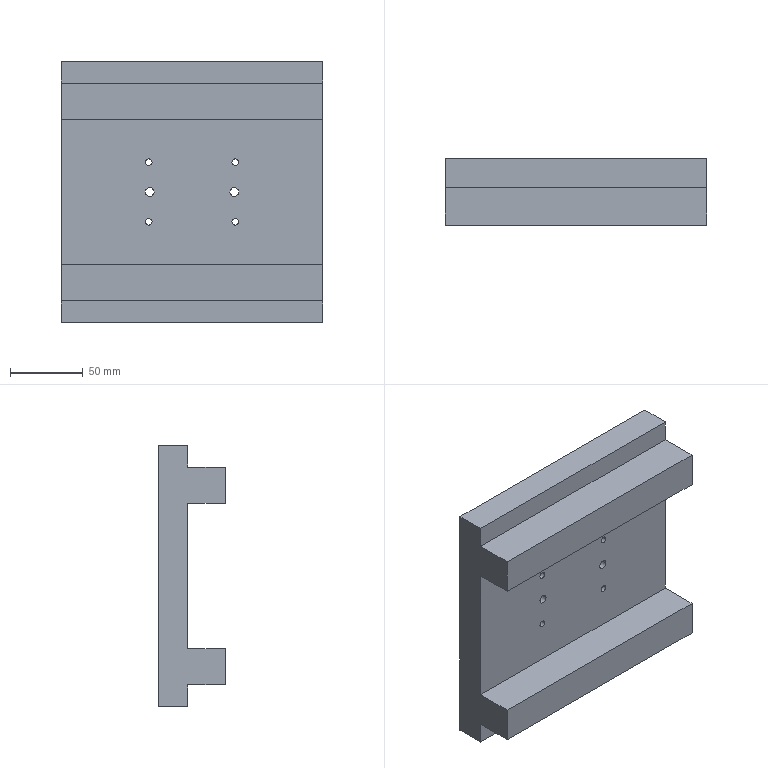Component | SolidWorks | WorkPlatform-1 | 1 solid | 41 faces | box 180 x 46 x 180 mm | volume 875888 mm3 | cylinder 22 | plane 19 | commonest cylinder face diameters 4.542 x8 8.034 x8 5.965 x4 16.633 x2
build123d program:
from build123d import *

# Parameters (mm, degrees)
SKETCH1_W           = 230
SKETCH1_H           = 230
BOSS_EXTRUDE1_DEPTH = 20
SKETCH3_R           = 4.017
CUT_EXTRUDE1_DEPTH  = 10
SKETCH4_R           = 2.271
CUT_EXTRUDE2_DEPTH  = 48
SKETCH5_R           = 2.983
CUT_EXTRUDE3_DEPTH  = 29
SKETCH6_W           = 24.865
SKETCH6_H           = 230
BOSS_EXTRUDE2_DEPTH = 26.003
SKETCH7_R           = 8.316
CUT_EXTRUDE4_DEPTH  = 1.5
SKETCH8_W           = 230
SKETCH8_H           = 230
SKETCH8_W_2         = 180
SKETCH8_H_2         = 180
CUT_EXTRUDE6_DEPTH  = 72
SKETCH9_R           = 8.316
CUT_EXTRUDE7_DEPTH  = 5


with BuildPart() as part:
    # Sketch1 → Boss-Extrude1 (new body)
    with BuildSketch(Plane(origin=(0, 0, 0), x_dir=(1, 0, 0), z_dir=(0, 1, 0))):
        Rectangle(SKETCH1_W, SKETCH1_H)
    extrude(amount=BOSS_EXTRUDE1_DEPTH)

    # Sketch3 → Cut-Extrude1 (cut)
    with BuildSketch(Plane(origin=(0, 20, 0), x_dir=(1, 0, 0), z_dir=(0, 1, 0))):
        with Locations(Location((20.473, 29.799, 0), (0, 0, 270))):
            Circle(SKETCH3_R)
        with Locations(Location((20.473, -29.799, 0), (0, 0, 90))):
            Circle(SKETCH3_R)
        with Locations(Location((-20.473, -29.799, 0), (0, 0, 270))):
            Circle(SKETCH3_R)
        with Locations(Location((-20.473, 29.799, 0), (0, 0, 90))):
            Circle(SKETCH3_R)
    extrude(amount=-CUT_EXTRUDE1_DEPTH, mode=Mode.SUBTRACT)

    # Sketch4 → Cut-Extrude2 (cut)
    with BuildSketch(Plane(origin=(0, 10, 0), x_dir=(1, 0, 0), z_dir=(0, 1, 0))):
        with Locations(Location((20.473, 29.799, 0), (0, 0, 270))):
            Circle(SKETCH4_R)
        with Locations(Location((20.473, -29.799, 0), (0, 0, 270))):
            Circle(SKETCH4_R)
        with Locations(Location((-20.473, -29.799, 0), (0, 0, 270))):
            Circle(SKETCH4_R)
        with Locations(Location((-20.473, 29.799, 0), (0, 0, 270))):
            Circle(SKETCH4_R)
    extrude(amount=-CUT_EXTRUDE2_DEPTH, mode=Mode.SUBTRACT)

    # Sketch5 → Cut-Extrude3 (cut)
    with BuildSketch(Plane(origin=(0, 20, 0), x_dir=(1, 0, 0), z_dir=(0, 1, 0))):
        with Locations(Location((0, 29.142, 0), (0, 0, 270))):
            Circle(SKETCH5_R)
        with Locations(Location((0, -29.142, 0), (0, 0, 270))):
            Circle(SKETCH5_R)
    extrude(amount=-CUT_EXTRUDE3_DEPTH, mode=Mode.SUBTRACT)

    # Sketch6 → Boss-Extrude2 (add)
    with BuildSketch(Plane.XZ):
        with Locations((-62.567, 0)):
            Rectangle(SKETCH6_W, SKETCH6_H)
    boss_extrude2 = extrude(amount=BOSS_EXTRUDE2_DEPTH)

    # Mirror1: Boss-Extrude2 across plane
    add(boss_extrude2.mirror(Plane.ZY))

    # Sketch7 → Cut-Extrude4 (cut)
    with BuildSketch(Plane.XY.offset(115)):
        with Locations((67.772, -0.5408)):
            Circle(SKETCH7_R)
    extrude(amount=-CUT_EXTRUDE4_DEPTH, mode=Mode.SUBTRACT)

    # Sketch8 → Cut-Extrude6 (cut)
    with BuildSketch(Plane(origin=(0, 20, 0), x_dir=(1, 0, 0), z_dir=(0, 1, 0))):
        Rectangle(SKETCH8_W, SKETCH8_H)
        Rectangle(SKETCH8_W_2, SKETCH8_H_2, mode=Mode.SUBTRACT)
    extrude(amount=-CUT_EXTRUDE6_DEPTH, mode=Mode.SUBTRACT)

    # Sketch9 → Cut-Extrude7 (cut)
    with BuildSketch(Plane.XY.offset(90)):
        with Locations((63.122, -0.688)):
            Circle(SKETCH9_R)
    extrude(amount=-CUT_EXTRUDE7_DEPTH, mode=Mode.SUBTRACT)


solid = part.part

# Placed as in the assembly
solid = solid.moved(Location((56.772, 96.74, 0), (0, 90, 0)))